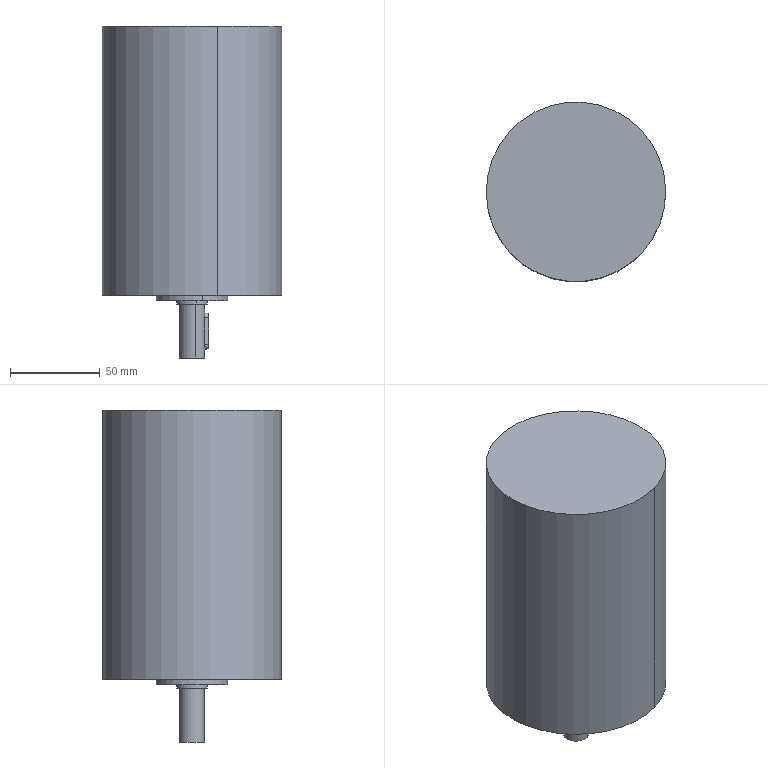Component | SolidWorks | DSEM-GDCServoGearMotor-1 | 1 solid | 35 faces | box 100 x 100 x 185 mm | volume 1186432 mm3 | cylinder 19 | cone 8 | plane 8 | commonest cylinder face diameters 4.2 x8 5 x3 40 x2 17 x2 100 x2 14 x2
build123d program:
from build123d import *

# Parameters (mm, degrees)
CIRPATTERN2_COUNT   = 4
BOSS_EXTRUDE1_DEPTH = 9


with BuildPart() as part:
    # Sketch1 → Revolve2 (revolve)
    with BuildSketch(Plane(origin=(0, 0, 0), x_dir=(0, 0, -1), z_dir=(1, 0, 0)), mode=Mode.PRIVATE) as revolve2_sk:
        Polygon((0, 20), (0, 50), (150, 50), (150, 0), (-35, 0), (-35, 7), (-5, 7), (-5, 8.5), (-3, 8.5), (-3, 20), align=None)
    revolve(revolve2_sk.sketch.rotate(Axis((0, 0, 38.169), (0, 0, -1)), 90), axis=Axis((0, 0, 38.169), (0, 0, -1)))

    # Sketch7 → M5 Tapped Hole2 (revolve, cut)
    with BuildSketch(Plane(origin=(-18.385, 18.385, 0), x_dir=(0, -1, 0), z_dir=(1, 0, 0))):
        Polygon((0, 0), (0, 13.662), (2.1, 12.4), (2.1, 0), align=None)
    m5_tapped_hole2 = revolve(axis=Axis((-18.385, 18.385, 6.35), (0, 0, -1)), mode=Mode.SUBTRACT)

    # CirPattern2: M5 Tapped Hole2 ×4 about axis
    cirpattern2_axis = Axis((0, 0, 0), (0, 0, 1))
    for i in range(1, CIRPATTERN2_COUNT):
        add(m5_tapped_hole2.rotate(cirpattern2_axis, i * 360 / CIRPATTERN2_COUNT), mode=Mode.SUBTRACT)

    # Sketch9 → Boss-Extrude1 (add)
    with BuildSketch(Plane(origin=(0, 0, 0), x_dir=(1, 0, 0), z_dir=(0, 1, 0))):
        with BuildLine():
            Line((2.5, -12.5), (2.5, -27.5))
            ThreePointArc((2.5, -27.5), (0, -30), (-2.5, -27.5))
            Line((-2.5, -27.5), (-2.5, -12.5))
            ThreePointArc((-2.5, -12.5), (0, -10), (2.5, -12.5))
        make_face()
    extrude(amount=BOSS_EXTRUDE1_DEPTH)


solid = part.part

# Placed as in the assembly
solid = solid.moved(Location((25.629, -64.9, 271), (-180, 0, -106.616)))
STEP:
#1=COLOUR_RGB('',0.7922,0.8196,0.9333);
#2=FILL_AREA_STYLE_COLOUR('',#1);
#3=FILL_AREA_STYLE('',(#2));
#4=SURFACE_STYLE_FILL_AREA(#3);
#5=SURFACE_SIDE_STYLE('',(#4));
#6=SURFACE_STYLE_USAGE(.BOTH.,#5);
#7=PRESENTATION_STYLE_ASSIGNMENT((#6));
#8=CARTESIAN_POINT('',(1.349,-2.454,10.276));
#9=VERTEX_POINT('',#8);
#10=CARTESIAN_POINT('',(1.377,-2.548,10.177));
#11=VERTEX_POINT('',#10);
#12=CARTESIAN_POINT('',(1.349,-2.454,10.177));
#13=DIRECTION('',(0.9582,0.286,-0.));
#14=DIRECTION('',(0.,0.,-1.));
#15=AXIS2_PLACEMENT_3D('',#12,#13,#14);
#16=CIRCLE('',#15,0.09843);
#17=EDGE_CURVE('',#9,#11,#16,.T.);
#18=ORIENTED_EDGE('',*,*,#17,.F.);
#19=CARTESIAN_POINT('',(1.273,-2.476,10.276));
#20=VERTEX_POINT('',#19);
#21=CARTESIAN_POINT('',(1.349,-2.454,10.276));
#22=DIRECTION('',(-0.9582,-0.286,0.));
#23=VECTOR('',#22,39.37);
#24=LINE('',#21,#23);
#25=EDGE_CURVE('',#9,#20,#24,.T.);
#26=ORIENTED_EDGE('',*,*,#25,.T.);
#27=CARTESIAN_POINT('',(1.284,-2.576,10.177));
#28=VERTEX_POINT('',#27);
#29=CARTESIAN_POINT('',(1.273,-2.476,10.276));
#30=CARTESIAN_POINT('',(1.275,-2.483,10.276));
#31=CARTESIAN_POINT('',(1.277,-2.489,10.275));
#32=CARTESIAN_POINT('',(1.279,-2.501,10.272));
#33=CARTESIAN_POINT('',(1.281,-2.507,10.27));
#34=CARTESIAN_POINT('',(1.282,-2.519,10.266));
#35=CARTESIAN_POINT('',(1.283,-2.525,10.262));
#36=CARTESIAN_POINT('',(1.284,-2.536,10.255));
#37=CARTESIAN_POINT('',(1.284,-2.541,10.251));
#38=CARTESIAN_POINT('',(1.285,-2.555,10.238));
#39=CARTESIAN_POINT('',(1.285,-2.563,10.227));
#40=CARTESIAN_POINT('',(1.284,-2.57,10.209));
#41=CARTESIAN_POINT('',(1.284,-2.572,10.203));
#42=CARTESIAN_POINT('',(1.284,-2.575,10.19));
#43=CARTESIAN_POINT('',(1.284,-2.576,10.184));
#44=CARTESIAN_POINT('',(1.284,-2.576,10.177));
#45=B_SPLINE_CURVE_WITH_KNOTS('',3,(#29,#30,#31,#32,#33,#34,#35,#36,#37,#38,#39,#40,#41,#42,#43,#44),.UNSPECIFIED.,.F.,.F.,(4,2,2,2,2,2,2,4),(0.,0.0004928,0.0009856,0.001478,0.001971,0.002957,0.003449,0.003942),.UNSPECIFIED.);
#46=EDGE_CURVE('',#20,#28,#45,.T.);
#47=ORIENTED_EDGE('',*,*,#46,.T.);
#48=CARTESIAN_POINT('',(1.377,-2.548,10.177));
#49=DIRECTION('',(-0.9582,-0.286,0.));
#50=VECTOR('',#49,39.37);
#51=LINE('',#48,#50);
#52=EDGE_CURVE('',#11,#28,#51,.T.);
#53=ORIENTED_EDGE('',*,*,#52,.F.);
#54=EDGE_LOOP('',(#18,#26,#47,#53));
#55=FACE_OUTER_BOUND('',#54,.T.);
#56=CARTESIAN_POINT('',(1.349,-2.454,10.177));
#57=DIRECTION('',(-0.9582,-0.286,0.));
#58=DIRECTION('',(0.,0.,1.));
#59=AXIS2_PLACEMENT_3D('',#56,#57,#58);
#60=CYLINDRICAL_SURFACE('',#59,0.09843);
#61=ADVANCED_FACE('',(#55),#60,.T.);
#62=CARTESIAN_POINT('',(0.5461,-3.535,11.157));
#63=VERTEX_POINT('',#62);
#64=CARTESIAN_POINT('',(0.4988,-3.376,11.157));
#65=VERTEX_POINT('',#64);
#66=CARTESIAN_POINT('',(0.5224,-3.456,11.157));
#67=DIRECTION('',(-0.,0.,-1.));
#68=DIRECTION('',(-0.286,0.9582,0.));
#69=AXIS2_PLACEMENT_3D('',#66,#67,#68);
#70=CIRCLE('',#69,0.08268);
#71=EDGE_CURVE('',#63,#65,#70,.T.);
#72=ORIENTED_EDGE('',*,*,#71,.F.);
#73=CARTESIAN_POINT('',(0.5461,-3.535,10.669));
#74=VERTEX_POINT('',#73);
#75=CARTESIAN_POINT('',(0.5461,-3.535,10.669));
#76=DIRECTION('',(-0.,0.,-1.));
#77=VECTOR('',#76,39.37);
#78=LINE('',#75,#77);
#79=EDGE_CURVE('',#63,#74,#78,.T.);
#80=ORIENTED_EDGE('',*,*,#79,.T.);
#81=CARTESIAN_POINT('',(0.4988,-3.376,10.669));
#82=VERTEX_POINT('',#81);
#83=CARTESIAN_POINT('',(0.5224,-3.456,10.669));
#84=DIRECTION('',(-0.,0.,-1.));
#85=DIRECTION('',(-0.286,0.9582,0.));
#86=AXIS2_PLACEMENT_3D('',#83,#84,#85);
#87=CIRCLE('',#86,0.08268);
#88=EDGE_CURVE('',#74,#82,#87,.T.);
#89=ORIENTED_EDGE('',*,*,#88,.T.);
#90=CARTESIAN_POINT('',(0.4988,-3.376,10.669));
#91=DIRECTION('',(-0.,0.,-1.));
#92=VECTOR('',#91,39.37);
#93=LINE('',#90,#92);
#94=EDGE_CURVE('',#65,#82,#93,.T.);
#95=ORIENTED_EDGE('',*,*,#94,.F.);
#96=EDGE_LOOP('',(#72,#80,#89,#95));
#97=FACE_OUTER_BOUND('',#96,.T.);
#98=CARTESIAN_POINT('',(0.5224,-3.456,10.669));
#99=DIRECTION('',(-0.,0.,-1.));
#100=DIRECTION('',(-0.286,0.9582,0.));
#101=AXIS2_PLACEMENT_3D('',#98,#99,#100);
#102=CYLINDRICAL_SURFACE('',#101,0.08268);
#103=ADVANCED_FACE('',(#97),#102,.F.);
#104=CARTESIAN_POINT('',(0.5224,-3.456,11.207));
#105=VERTEX_POINT('',#104);
#106=CARTESIAN_POINT('',(0.4988,-3.376,11.157));
#107=DIRECTION('',(-0.2451,0.8214,-0.515));
#108=VECTOR('',#107,39.37);
#109=LINE('',#106,#108);
#110=EDGE_CURVE('',#105,#65,#109,.T.);
#111=ORIENTED_EDGE('',*,*,#110,.F.);
#112=CARTESIAN_POINT('',(0.5461,-3.535,11.157));
#113=DIRECTION('',(0.2451,-0.8214,-0.515));
#114=VECTOR('',#113,39.37);
#115=LINE('',#112,#114);
#116=EDGE_CURVE('',#105,#63,#115,.T.);
#117=ORIENTED_EDGE('',*,*,#116,.T.);
#118=ORIENTED_EDGE('',*,*,#71,.T.);
#119=EDGE_LOOP('',(#111,#117,#118));
#120=FACE_OUTER_BOUND('',#119,.T.);
#121=CARTESIAN_POINT('',(0.5224,-3.456,11.157));
#122=DIRECTION('',(-0.,0.,-1.));
#123=DIRECTION('',(-0.286,0.9582,0.));
#124=AXIS2_PLACEMENT_3D('',#121,#122,#123);
#125=CONICAL_SURFACE('',#124,0.08268,1.03);
#126=ADVANCED_FACE('',(#120),#125,.F.);
#127=CARTESIAN_POINT('',(0.1321,-2.148,11.157));
#128=VERTEX_POINT('',#127);
#129=CARTESIAN_POINT('',(0.08483,-1.989,11.157));
#130=VERTEX_POINT('',#129);
#131=CARTESIAN_POINT('',(0.1085,-2.069,11.157));
#132=DIRECTION('',(-0.,0.,-1.));
#133=DIRECTION('',(-0.286,0.9582,0.));
#134=AXIS2_PLACEMENT_3D('',#131,#132,#133);
#135=CIRCLE('',#134,0.08268);
#136=EDGE_CURVE('',#128,#130,#135,.T.);
#137=ORIENTED_EDGE('',*,*,#136,.F.);
#138=CARTESIAN_POINT('',(0.1321,-2.148,10.669));
#139=VERTEX_POINT('',#138);
#140=CARTESIAN_POINT('',(0.1321,-2.148,10.669));
#141=DIRECTION('',(-0.,0.,-1.));
#142=VECTOR('',#141,39.37);
#143=LINE('',#140,#142);
#144=EDGE_CURVE('',#128,#139,#143,.T.);
#145=ORIENTED_EDGE('',*,*,#144,.T.);
#146=CARTESIAN_POINT('',(0.08483,-1.989,10.669));
#147=VERTEX_POINT('',#146);
#148=CARTESIAN_POINT('',(0.1085,-2.069,10.669));
#149=DIRECTION('',(-0.,0.,-1.));
#150=DIRECTION('',(-0.286,0.9582,0.));
#151=AXIS2_PLACEMENT_3D('',#148,#149,#150);
#152=CIRCLE('',#151,0.08268);
#153=EDGE_CURVE('',#139,#147,#152,.T.);
#154=ORIENTED_EDGE('',*,*,#153,.T.);
#155=CARTESIAN_POINT('',(0.08483,-1.989,10.669));
#156=DIRECTION('',(-0.,0.,-1.));
#157=VECTOR('',#156,39.37);
#158=LINE('',#155,#157);
#159=EDGE_CURVE('',#130,#147,#158,.T.);
#160=ORIENTED_EDGE('',*,*,#159,.F.);
#161=EDGE_LOOP('',(#137,#145,#154,#160));
#162=FACE_OUTER_BOUND('',#161,.T.);
#163=CARTESIAN_POINT('',(0.1085,-2.069,10.669));
#164=DIRECTION('',(-0.,0.,-1.));
#165=DIRECTION('',(-0.286,0.9582,0.));
#166=AXIS2_PLACEMENT_3D('',#163,#164,#165);
#167=CYLINDRICAL_SURFACE('',#166,0.08268);
#168=ADVANCED_FACE('',(#162),#167,.F.);
#169=CARTESIAN_POINT('',(0.1085,-2.069,11.207));
#170=VERTEX_POINT('',#169);
#171=CARTESIAN_POINT('',(0.08483,-1.989,11.157));
#172=DIRECTION('',(-0.2451,0.8214,-0.515));
#173=VECTOR('',#172,39.37);
#174=LINE('',#171,#173);
#175=EDGE_CURVE('',#170,#130,#174,.T.);
#176=ORIENTED_EDGE('',*,*,#175,.F.);
#177=CARTESIAN_POINT('',(0.1321,-2.148,11.157));
#178=DIRECTION('',(0.2451,-0.8214,-0.515));
#179=VECTOR('',#178,39.37);
#180=LINE('',#177,#179);
#181=EDGE_CURVE('',#170,#128,#180,.T.);
#182=ORIENTED_EDGE('',*,*,#181,.T.);
#183=ORIENTED_EDGE('',*,*,#136,.T.);
#184=EDGE_LOOP('',(#176,#182,#183));
#185=FACE_OUTER_BOUND('',#184,.T.);
#186=CARTESIAN_POINT('',(0.1085,-2.069,11.157));
#187=DIRECTION('',(-0.,0.,-1.));
#188=DIRECTION('',(-0.286,0.9582,0.));
#189=AXIS2_PLACEMENT_3D('',#186,#187,#188);
#190=CONICAL_SURFACE('',#189,0.08268,1.03);
#191=ADVANCED_FACE('',(#185),#190,.F.);
#192=CARTESIAN_POINT('',(1.519,-1.734,11.157));
#193=VERTEX_POINT('',#192);
#194=CARTESIAN_POINT('',(1.472,-1.575,11.157));
#195=VERTEX_POINT('',#194);
#196=CARTESIAN_POINT('',(1.496,-1.655,11.157));
#197=DIRECTION('',(-0.,0.,-1.));
#198=DIRECTION('',(-0.286,0.9582,0.));
#199=AXIS2_PLACEMENT_3D('',#196,#197,#198);
#200=CIRCLE('',#199,0.08268);
#201=EDGE_CURVE('',#193,#195,#200,.T.);
#202=ORIENTED_EDGE('',*,*,#201,.F.);
#203=CARTESIAN_POINT('',(1.519,-1.734,10.669));
#204=VERTEX_POINT('',#203);
#205=CARTESIAN_POINT('',(1.519,-1.734,10.669));
#206=DIRECTION('',(-0.,0.,-1.));
#207=VECTOR('',#206,39.37);
#208=LINE('',#205,#207);
#209=EDGE_CURVE('',#193,#204,#208,.T.);
#210=ORIENTED_EDGE('',*,*,#209,.T.);
#211=CARTESIAN_POINT('',(1.472,-1.575,10.669));
#212=VERTEX_POINT('',#211);
#213=CARTESIAN_POINT('',(1.496,-1.655,10.669));
#214=DIRECTION('',(-0.,0.,-1.));
#215=DIRECTION('',(-0.286,0.9582,0.));
#216=AXIS2_PLACEMENT_3D('',#213,#214,#215);
#217=CIRCLE('',#216,0.08268);
#218=EDGE_CURVE('',#204,#212,#217,.T.);
#219=ORIENTED_EDGE('',*,*,#218,.T.);
#220=CARTESIAN_POINT('',(1.472,-1.575,10.669));
#221=DIRECTION('',(-0.,0.,-1.));
#222=VECTOR('',#221,39.37);
#223=LINE('',#220,#222);
#224=EDGE_CURVE('',#195,#212,#223,.T.);
#225=ORIENTED_EDGE('',*,*,#224,.F.);
#226=EDGE_LOOP('',(#202,#210,#219,#225));
#227=FACE_OUTER_BOUND('',#226,.T.);
#228=CARTESIAN_POINT('',(1.496,-1.655,10.669));
#229=DIRECTION('',(-0.,0.,-1.));
#230=DIRECTION('',(-0.286,0.9582,0.));
#231=AXIS2_PLACEMENT_3D('',#228,#229,#230);
#232=CYLINDRICAL_SURFACE('',#231,0.08268);
#233=ADVANCED_FACE('',(#227),#232,.F.);
#234=CARTESIAN_POINT('',(1.496,-1.655,11.207));
#235=VERTEX_POINT('',#234);
#236=CARTESIAN_POINT('',(1.472,-1.575,11.157));
#237=DIRECTION('',(-0.2451,0.8214,-0.515));
#238=VECTOR('',#237,39.37);
#239=LINE('',#236,#238);
#240=EDGE_CURVE('',#235,#195,#239,.T.);
#241=ORIENTED_EDGE('',*,*,#240,.F.);
#242=CARTESIAN_POINT('',(1.519,-1.734,11.157));
#243=DIRECTION('',(0.2451,-0.8214,-0.515));
#244=VECTOR('',#243,39.37);
#245=LINE('',#242,#244);
#246=EDGE_CURVE('',#235,#193,#245,.T.);
#247=ORIENTED_EDGE('',*,*,#246,.T.);
#248=ORIENTED_EDGE('',*,*,#201,.T.);
#249=EDGE_LOOP('',(#241,#247,#248));
#250=FACE_OUTER_BOUND('',#249,.T.);
#251=CARTESIAN_POINT('',(1.496,-1.655,11.157));
#252=DIRECTION('',(-0.,0.,-1.));
#253=DIRECTION('',(-0.286,0.9582,0.));
#254=AXIS2_PLACEMENT_3D('',#251,#252,#253);
#255=CONICAL_SURFACE('',#254,0.08268,1.03);
#256=ADVANCED_FACE('',(#250),#255,.F.);
#257=CARTESIAN_POINT('',(1.933,-3.121,11.157));
#258=VERTEX_POINT('',#257);
#259=CARTESIAN_POINT('',(1.886,-2.963,11.157));
#260=VERTEX_POINT('',#259);
#261=CARTESIAN_POINT('',(1.91,-3.042,11.157));
#262=DIRECTION('',(-0.,0.,-1.));
#263=DIRECTION('',(-0.286,0.9582,0.));
#264=AXIS2_PLACEMENT_3D('',#261,#262,#263);
#265=CIRCLE('',#264,0.08268);
#266=EDGE_CURVE('',#258,#260,#265,.T.);
#267=ORIENTED_EDGE('',*,*,#266,.F.);
#268=CARTESIAN_POINT('',(1.933,-3.121,10.669));
#269=VERTEX_POINT('',#268);
#270=CARTESIAN_POINT('',(1.933,-3.121,10.669));
#271=DIRECTION('',(-0.,0.,-1.));
#272=VECTOR('',#271,39.37);
#273=LINE('',#270,#272);
#274=EDGE_CURVE('',#258,#269,#273,.T.);
#275=ORIENTED_EDGE('',*,*,#274,.T.);
#276=CARTESIAN_POINT('',(1.886,-2.963,10.669));
#277=VERTEX_POINT('',#276);
#278=CARTESIAN_POINT('',(1.91,-3.042,10.669));
#279=DIRECTION('',(-0.,0.,-1.));
#280=DIRECTION('',(-0.286,0.9582,0.));
#281=AXIS2_PLACEMENT_3D('',#278,#279,#280);
#282=CIRCLE('',#281,0.08268);
#283=EDGE_CURVE('',#269,#277,#282,.T.);
#284=ORIENTED_EDGE('',*,*,#283,.T.);
#285=CARTESIAN_POINT('',(1.886,-2.963,10.669));
#286=DIRECTION('',(-0.,0.,-1.));
#287=VECTOR('',#286,39.37);
#288=LINE('',#285,#287);
#289=EDGE_CURVE('',#260,#277,#288,.T.);
#290=ORIENTED_EDGE('',*,*,#289,.F.);
#291=EDGE_LOOP('',(#267,#275,#284,#290));
#292=FACE_OUTER_BOUND('',#291,.T.);
#293=CARTESIAN_POINT('',(1.91,-3.042,10.669));
#294=DIRECTION('',(-0.,0.,-1.));
#295=DIRECTION('',(-0.286,0.9582,0.));
#296=AXIS2_PLACEMENT_3D('',#293,#294,#295);
#297=CYLINDRICAL_SURFACE('',#296,0.08268);
#298=ADVANCED_FACE('',(#292),#297,.F.);
#299=CARTESIAN_POINT('',(1.91,-3.042,11.207));
#300=VERTEX_POINT('',#299);
#301=CARTESIAN_POINT('',(1.886,-2.963,11.157));
#302=DIRECTION('',(-0.2451,0.8214,-0.515));
#303=VECTOR('',#302,39.37);
#304=LINE('',#301,#303);
#305=EDGE_CURVE('',#300,#260,#304,.T.);
#306=ORIENTED_EDGE('',*,*,#305,.F.);
#307=CARTESIAN_POINT('',(1.933,-3.121,11.157));
#308=DIRECTION('',(0.2451,-0.8214,-0.515));
#309=VECTOR('',#308,39.37);
#310=LINE('',#307,#309);
#311=EDGE_CURVE('',#300,#258,#310,.T.);
#312=ORIENTED_EDGE('',*,*,#311,.T.);
#313=ORIENTED_EDGE('',*,*,#266,.T.);
#314=EDGE_LOOP('',(#306,#312,#313));
#315=FACE_OUTER_BOUND('',#314,.T.);
#316=CARTESIAN_POINT('',(1.91,-3.042,11.157));
#317=DIRECTION('',(-0.,0.,-1.));
#318=DIRECTION('',(-0.286,0.9582,0.));
#319=AXIS2_PLACEMENT_3D('',#316,#317,#318);
#320=CONICAL_SURFACE('',#319,0.08268,1.03);
#321=ADVANCED_FACE('',(#315),#320,.F.);
#322=CARTESIAN_POINT('',(0.7839,-1.801,10.669));
#323=VERTEX_POINT('',#322);
#324=CARTESIAN_POINT('',(1.234,-3.31,10.669));
#325=VERTEX_POINT('',#324);
#326=CARTESIAN_POINT('',(1.009,-2.555,10.669));
#327=DIRECTION('',(-0.,0.,-1.));
#328=DIRECTION('',(-0.286,0.9582,0.));
#329=AXIS2_PLACEMENT_3D('',#326,#327,#328);
#330=CIRCLE('',#329,0.7874);
#331=EDGE_CURVE('',#323,#325,#330,.T.);
#332=ORIENTED_EDGE('',*,*,#331,.T.);
#333=CARTESIAN_POINT('',(1.234,-3.31,10.551));
#334=VERTEX_POINT('',#333);
#335=CARTESIAN_POINT('',(1.234,-3.31,9.167));
#336=DIRECTION('',(-0.,0.,-1.));
#337=VECTOR('',#336,39.37);
#338=LINE('',#335,#337);
#339=EDGE_CURVE('',#325,#334,#338,.T.);
#340=ORIENTED_EDGE('',*,*,#339,.T.);
#341=CARTESIAN_POINT('',(0.7839,-1.801,10.551));
#342=VERTEX_POINT('',#341);
#343=CARTESIAN_POINT('',(1.009,-2.555,10.551));
#344=DIRECTION('',(-0.,0.,-1.));
#345=DIRECTION('',(-0.286,0.9582,0.));
#346=AXIS2_PLACEMENT_3D('',#343,#344,#345);
#347=CIRCLE('',#346,0.7874);
#348=EDGE_CURVE('',#342,#334,#347,.T.);
#349=ORIENTED_EDGE('',*,*,#348,.F.);
#350=CARTESIAN_POINT('',(0.7839,-1.801,9.167));
#351=DIRECTION('',(-0.,0.,-1.));
#352=VECTOR('',#351,39.37);
#353=LINE('',#350,#352);
#354=EDGE_CURVE('',#323,#342,#353,.T.);
#355=ORIENTED_EDGE('',*,*,#354,.F.);
#356=EDGE_LOOP('',(#332,#340,#349,#355));
#357=FACE_OUTER_BOUND('',#356,.T.);
#358=CARTESIAN_POINT('',(1.009,-2.555,9.167));
#359=DIRECTION('',(-0.,0.,-1.));
#360=DIRECTION('',(-0.286,0.9582,0.));
#361=AXIS2_PLACEMENT_3D('',#358,#359,#360);
#362=CYLINDRICAL_SURFACE('',#361,0.7874);
#363=ADVANCED_FACE('',(#357),#362,.T.);
#364=CARTESIAN_POINT('',(0.9133,-2.234,10.551));
#365=VERTEX_POINT('',#364);
#366=CARTESIAN_POINT('',(1.105,-2.876,10.551));
#367=VERTEX_POINT('',#366);
#368=CARTESIAN_POINT('',(1.009,-2.555,10.551));
#369=DIRECTION('',(-0.,0.,-1.));
#370=DIRECTION('',(-0.286,0.9582,0.));
#371=AXIS2_PLACEMENT_3D('',#368,#369,#370);
#372=CIRCLE('',#371,0.3346);
#373=EDGE_CURVE('',#365,#367,#372,.T.);
#374=ORIENTED_EDGE('',*,*,#373,.T.);
#375=CARTESIAN_POINT('',(1.105,-2.876,10.472));
#376=VERTEX_POINT('',#375);
#377=CARTESIAN_POINT('',(1.105,-2.876,9.167));
#378=DIRECTION('',(-0.,0.,-1.));
#379=VECTOR('',#378,39.37);
#380=LINE('',#377,#379);
#381=EDGE_CURVE('',#367,#376,#380,.T.);
#382=ORIENTED_EDGE('',*,*,#381,.T.);
#383=CARTESIAN_POINT('',(0.9133,-2.234,10.472));
#384=VERTEX_POINT('',#383);
#385=CARTESIAN_POINT('',(1.009,-2.555,10.472));
#386=DIRECTION('',(-0.,0.,-1.));
#387=DIRECTION('',(-0.286,0.9582,0.));
#388=AXIS2_PLACEMENT_3D('',#385,#386,#387);
#389=CIRCLE('',#388,0.3346);
#390=EDGE_CURVE('',#384,#376,#389,.T.);
#391=ORIENTED_EDGE('',*,*,#390,.F.);
#392=CARTESIAN_POINT('',(0.9133,-2.234,9.167));
#393=DIRECTION('',(-0.,0.,-1.));
#394=VECTOR('',#393,39.37);
#395=LINE('',#392,#394);
#396=EDGE_CURVE('',#365,#384,#395,.T.);
#397=ORIENTED_EDGE('',*,*,#396,.F.);
#398=EDGE_LOOP('',(#374,#382,#391,#397));
#399=FACE_OUTER_BOUND('',#398,.T.);
#400=CARTESIAN_POINT('',(1.009,-2.555,9.167));
#401=DIRECTION('',(-0.,0.,-1.));
#402=DIRECTION('',(-0.286,0.9582,0.));
#403=AXIS2_PLACEMENT_3D('',#400,#401,#402);
#404=CYLINDRICAL_SURFACE('',#403,0.3346);
#405=ADVANCED_FACE('',(#399),#404,.T.);
#406=CARTESIAN_POINT('',(0.4461,-0.6688,16.575));
#407=VERTEX_POINT('',#406);
#408=CARTESIAN_POINT('',(1.572,-4.441,16.575));
#409=VERTEX_POINT('',#408);
#410=CARTESIAN_POINT('',(1.009,-2.555,16.575));
#411=DIRECTION('',(-0.,0.,-1.));
#412=DIRECTION('',(-0.286,0.9582,0.));
#413=AXIS2_PLACEMENT_3D('',#410,#411,#412);
#414=CIRCLE('',#413,1.969);
#415=EDGE_CURVE('',#407,#409,#414,.T.);
#416=ORIENTED_EDGE('',*,*,#415,.T.);
#417=CARTESIAN_POINT('',(1.572,-4.441,10.669));
#418=VERTEX_POINT('',#417);
#419=CARTESIAN_POINT('',(1.572,-4.441,9.167));
#420=DIRECTION('',(-0.,0.,-1.));
#421=VECTOR('',#420,39.37);
#422=LINE('',#419,#421);
#423=EDGE_CURVE('',#409,#418,#422,.T.);
#424=ORIENTED_EDGE('',*,*,#423,.T.);
#425=CARTESIAN_POINT('',(0.4461,-0.6688,10.669));
#426=VERTEX_POINT('',#425);
#427=CARTESIAN_POINT('',(1.009,-2.555,10.669));
#428=DIRECTION('',(-0.,0.,-1.));
#429=DIRECTION('',(-0.286,0.9582,0.));
#430=AXIS2_PLACEMENT_3D('',#427,#428,#429);
#431=CIRCLE('',#430,1.969);
#432=EDGE_CURVE('',#426,#418,#431,.T.);
#433=ORIENTED_EDGE('',*,*,#432,.F.);
#434=CARTESIAN_POINT('',(0.4461,-0.6688,9.167));
#435=DIRECTION('',(-0.,0.,-1.));
#436=VECTOR('',#435,39.37);
#437=LINE('',#434,#436);
#438=EDGE_CURVE('',#407,#426,#437,.T.);
#439=ORIENTED_EDGE('',*,*,#438,.F.);
#440=EDGE_LOOP('',(#416,#424,#433,#439));
#441=FACE_OUTER_BOUND('',#440,.T.);
#442=CARTESIAN_POINT('',(1.009,-2.555,9.167));
#443=DIRECTION('',(-0.,0.,-1.));
#444=DIRECTION('',(-0.286,0.9582,0.));
#445=AXIS2_PLACEMENT_3D('',#442,#443,#444);
#446=CYLINDRICAL_SURFACE('',#445,1.969);
#447=ADVANCED_FACE('',(#441),#446,.T.);
#448=CARTESIAN_POINT('',(1.228,-2.387,10.177));
#449=VERTEX_POINT('',#448);
#450=CARTESIAN_POINT('',(1.228,-2.387,10.177));
#451=CARTESIAN_POINT('',(1.228,-2.387,10.184));
#452=CARTESIAN_POINT('',(1.228,-2.388,10.19));
#453=CARTESIAN_POINT('',(1.23,-2.39,10.203));
#454=CARTESIAN_POINT('',(1.231,-2.392,10.209));
#455=CARTESIAN_POINT('',(1.234,-2.396,10.221));
#456=CARTESIAN_POINT('',(1.236,-2.398,10.227));
#457=CARTESIAN_POINT('',(1.24,-2.405,10.237));
#458=CARTESIAN_POINT('',(1.242,-2.408,10.242));
#459=CARTESIAN_POINT('',(1.247,-2.416,10.251));
#460=CARTESIAN_POINT('',(1.25,-2.421,10.255));
#461=CARTESIAN_POINT('',(1.255,-2.43,10.263));
#462=CARTESIAN_POINT('',(1.257,-2.435,10.266));
#463=CARTESIAN_POINT('',(1.262,-2.446,10.271));
#464=CARTESIAN_POINT('',(1.265,-2.452,10.272));
#465=CARTESIAN_POINT('',(1.269,-2.464,10.275));
#466=CARTESIAN_POINT('',(1.271,-2.47,10.276));
#467=CARTESIAN_POINT('',(1.273,-2.476,10.276));
#468=B_SPLINE_CURVE_WITH_KNOTS('',3,(#450,#451,#452,#453,#454,#455,#456,#457,#458,#459,#460,#461,#462,#463,#464,#465,#466,#467),.UNSPECIFIED.,.F.,.F.,(4,2,2,2,2,2,2,2,4),(0.01182,0.01231,0.01281,0.0133,0.01379,0.01428,0.01478,0.01527,0.01576),.UNSPECIFIED.);
#469=EDGE_CURVE('',#449,#20,#468,.T.);
#470=ORIENTED_EDGE('',*,*,#469,.F.);
#471=CARTESIAN_POINT('',(1.228,-2.387,9.587));
#472=VERTEX_POINT('',#471);
#473=CARTESIAN_POINT('',(1.228,-2.387,9.167));
#474=DIRECTION('',(0.,-0.,1.));
#475=VECTOR('',#474,39.37);
#476=LINE('',#473,#475);
#477=EDGE_CURVE('',#472,#449,#476,.T.);
#478=ORIENTED_EDGE('',*,*,#477,.F.);
#479=CARTESIAN_POINT('',(1.284,-2.576,9.587));
#480=VERTEX_POINT('',#479);
#481=CARTESIAN_POINT('',(1.284,-2.576,9.587));
#482=CARTESIAN_POINT('',(1.284,-2.576,9.58));
#483=CARTESIAN_POINT('',(1.284,-2.575,9.574));
#484=CARTESIAN_POINT('',(1.284,-2.572,9.561));
#485=CARTESIAN_POINT('',(1.284,-2.57,9.555));
#486=CARTESIAN_POINT('',(1.284,-2.565,9.543));
#487=CARTESIAN_POINT('',(1.285,-2.562,9.537));
#488=CARTESIAN_POINT('',(1.285,-2.554,9.526));
#489=CARTESIAN_POINT('',(1.285,-2.55,9.521));
#490=CARTESIAN_POINT('',(1.284,-2.541,9.512));
#491=CARTESIAN_POINT('',(1.284,-2.536,9.508));
#492=CARTESIAN_POINT('',(1.283,-2.525,9.501));
#493=CARTESIAN_POINT('',(1.282,-2.519,9.498));
#494=CARTESIAN_POINT('',(1.281,-2.507,9.493));
#495=CARTESIAN_POINT('',(1.279,-2.501,9.491));
#496=CARTESIAN_POINT('',(1.277,-2.489,9.489));
#497=CARTESIAN_POINT('',(1.275,-2.483,9.488));
#498=CARTESIAN_POINT('',(1.271,-2.47,9.488));
#499=CARTESIAN_POINT('',(1.269,-2.464,9.489));
#500=CARTESIAN_POINT('',(1.265,-2.452,9.491));
#501=CARTESIAN_POINT('',(1.262,-2.446,9.493));
#502=CARTESIAN_POINT('',(1.257,-2.435,9.498));
#503=CARTESIAN_POINT('',(1.255,-2.43,9.501));
#504=CARTESIAN_POINT('',(1.25,-2.421,9.508));
#505=CARTESIAN_POINT('',(1.247,-2.416,9.512));
#506=CARTESIAN_POINT('',(1.242,-2.408,9.522));
#507=CARTESIAN_POINT('',(1.24,-2.405,9.527));
#508=CARTESIAN_POINT('',(1.236,-2.398,9.537));
#509=CARTESIAN_POINT('',(1.234,-2.396,9.543));
#510=CARTESIAN_POINT('',(1.231,-2.392,9.555));
#511=CARTESIAN_POINT('',(1.23,-2.39,9.561));
#512=CARTESIAN_POINT('',(1.228,-2.388,9.574));
#513=CARTESIAN_POINT('',(1.228,-2.387,9.58));
#514=CARTESIAN_POINT('',(1.228,-2.387,9.587));
#515=B_SPLINE_CURVE_WITH_KNOTS('',3,(#481,#482,#483,#484,#485,#486,#487,#488,#489,#490,#491,#492,#493,#494,#495,#496,#497,#498,#499,#500,#501,#502,#503,#504,#505,#506,#507,#508,#509,#510,#511,#512,#513,#514),.UNSPECIFIED.,.F.,.F.,(4,2,2,2,2,2,2,2,2,2,2,2,2,2,2,2,4),(0.003942,0.004435,0.004927,0.005419,0.005912,0.006404,0.006897,0.007389,0.007882,0.008374,0.008866,0.009359,0.009851,0.01034,0.01084,0.01133,0.01182),.UNSPECIFIED.);
#516=EDGE_CURVE('',#480,#472,#515,.T.);
#517=ORIENTED_EDGE('',*,*,#516,.F.);
#518=CARTESIAN_POINT('',(1.284,-2.576,9.167));
#519=DIRECTION('',(-0.,0.,-1.));
#520=VECTOR('',#519,39.37);
#521=LINE('',#518,#520);
#522=EDGE_CURVE('',#28,#480,#521,.T.);
#523=ORIENTED_EDGE('',*,*,#522,.F.);
#524=ORIENTED_EDGE('',*,*,#46,.F.);
#525=EDGE_LOOP('',(#470,#478,#517,#523,#524));
#526=FACE_BOUND('',#525,.T.);
#527=CARTESIAN_POINT('',(0.9302,-2.291,10.472));
#528=VERTEX_POINT('',#527);
#529=CARTESIAN_POINT('',(1.088,-2.819,10.472));
#530=VERTEX_POINT('',#529);
#531=CARTESIAN_POINT('',(1.009,-2.555,10.472));
#532=DIRECTION('',(-0.,0.,-1.));
#533=DIRECTION('',(-0.286,0.9582,0.));
#534=AXIS2_PLACEMENT_3D('',#531,#532,#533);
#535=CIRCLE('',#534,0.2756);
#536=EDGE_CURVE('',#528,#530,#535,.T.);
#537=ORIENTED_EDGE('',*,*,#536,.T.);
#538=CARTESIAN_POINT('',(1.088,-2.819,9.291));
#539=VERTEX_POINT('',#538);
#540=CARTESIAN_POINT('',(1.088,-2.819,9.167));
#541=DIRECTION('',(-0.,0.,-1.));
#542=VECTOR('',#541,39.37);
#543=LINE('',#540,#542);
#544=EDGE_CURVE('',#530,#539,#543,.T.);
#545=ORIENTED_EDGE('',*,*,#544,.T.);
#546=CARTESIAN_POINT('',(0.9302,-2.291,9.291));
#547=VERTEX_POINT('',#546);
#548=CARTESIAN_POINT('',(1.009,-2.555,9.291));
#549=DIRECTION('',(-0.,0.,-1.));
#550=DIRECTION('',(-0.286,0.9582,0.));
#551=AXIS2_PLACEMENT_3D('',#548,#549,#550);
#552=CIRCLE('',#551,0.2756);
#553=EDGE_CURVE('',#547,#539,#552,.T.);
#554=ORIENTED_EDGE('',*,*,#553,.F.);
#555=CARTESIAN_POINT('',(0.9302,-2.291,9.167));
#556=DIRECTION('',(-0.,0.,-1.));
#557=VECTOR('',#556,39.37);
#558=LINE('',#555,#557);
#559=EDGE_CURVE('',#528,#547,#558,.T.);
#560=ORIENTED_EDGE('',*,*,#559,.F.);
#561=EDGE_LOOP('',(#537,#545,#554,#560));
#562=FACE_OUTER_BOUND('',#561,.T.);
#563=CARTESIAN_POINT('',(1.009,-2.555,9.167));
#564=DIRECTION('',(-0.,0.,-1.));
#565=DIRECTION('',(-0.286,0.9582,0.));
#566=AXIS2_PLACEMENT_3D('',#563,#564,#565);
#567=CYLINDRICAL_SURFACE('',#566,0.2756);
#568=ADVANCED_FACE('',(#526,#562),#567,.T.);
#569=ORIENTED_EDGE('',*,*,#544,.F.);
#570=CARTESIAN_POINT('',(1.009,-2.555,10.472));
#571=DIRECTION('',(-0.,0.,-1.));
#572=DIRECTION('',(-0.286,0.9582,0.));
#573=AXIS2_PLACEMENT_3D('',#570,#571,#572);
#574=CIRCLE('',#573,0.2756);
#575=EDGE_CURVE('',#530,#528,#574,.T.);
#576=ORIENTED_EDGE('',*,*,#575,.T.);
#577=ORIENTED_EDGE('',*,*,#559,.T.);
#578=CARTESIAN_POINT('',(1.009,-2.555,9.291));
#579=DIRECTION('',(-0.,0.,-1.));
#580=DIRECTION('',(-0.286,0.9582,0.));
#581=AXIS2_PLACEMENT_3D('',#578,#579,#580);
#582=CIRCLE('',#581,0.2756);
#583=EDGE_CURVE('',#539,#547,#582,.T.);
#584=ORIENTED_EDGE('',*,*,#583,.F.);
#585=EDGE_LOOP('',(#569,#576,#577,#584));
#586=FACE_OUTER_BOUND('',#585,.T.);
#587=CARTESIAN_POINT('',(1.009,-2.555,9.167));
#588=DIRECTION('',(-0.,0.,-1.));
#589=DIRECTION('',(-0.286,0.9582,0.));
#590=AXIS2_PLACEMENT_3D('',#587,#588,#589);
#591=CYLINDRICAL_SURFACE('',#590,0.2756);
#592=ADVANCED_FACE('',(#586),#591,.T.);
#593=ORIENTED_EDGE('',*,*,#423,.F.);
#594=CARTESIAN_POINT('',(1.009,-2.555,16.575));
#595=DIRECTION('',(-0.,0.,-1.));
#596=DIRECTION('',(-0.286,0.9582,0.));
#597=AXIS2_PLACEMENT_3D('',#594,#595,#596);
#598=CIRCLE('',#597,1.969);
#599=EDGE_CURVE('',#409,#407,#598,.T.);
#600=ORIENTED_EDGE('',*,*,#599,.T.);
#601=ORIENTED_EDGE('',*,*,#438,.T.);
#602=CARTESIAN_POINT('',(1.009,-2.555,10.669));
#603=DIRECTION('',(-0.,0.,-1.));
#604=DIRECTION('',(-0.286,0.9582,0.));
#605=AXIS2_PLACEMENT_3D('',#602,#603,#604);
#606=CIRCLE('',#605,1.969);
#607=EDGE_CURVE('',#418,#426,#606,.T.);
#608=ORIENTED_EDGE('',*,*,#607,.F.);
#609=EDGE_LOOP('',(#593,#600,#601,#608));
#610=FACE_OUTER_BOUND('',#609,.T.);
#611=CARTESIAN_POINT('',(1.009,-2.555,9.167));
#612=DIRECTION('',(-0.,0.,-1.));
#613=DIRECTION('',(-0.286,0.9582,0.));
#614=AXIS2_PLACEMENT_3D('',#611,#612,#613);
#615=CYLINDRICAL_SURFACE('',#614,1.969);
#616=ADVANCED_FACE('',(#610),#615,.T.);
#617=ORIENTED_EDGE('',*,*,#415,.F.);
#618=ORIENTED_EDGE('',*,*,#599,.F.);
#619=EDGE_LOOP('',(#617,#618));
#620=FACE_OUTER_BOUND('',#619,.T.);
#621=CARTESIAN_POINT('',(2.895,-1.992,16.575));
#622=DIRECTION('',(-0.,0.,-1.));
#623=DIRECTION('',(-0.286,0.9582,0.));
#624=AXIS2_PLACEMENT_3D('',#621,#622,#623);
#625=PLANE('',#624);
#626=ADVANCED_FACE('',(#620),#625,.F.);
#627=ORIENTED_EDGE('',*,*,#553,.T.);
#628=ORIENTED_EDGE('',*,*,#583,.T.);
#629=EDGE_LOOP('',(#627,#628));
#630=FACE_OUTER_BOUND('',#629,.T.);
#631=CARTESIAN_POINT('',(1.273,-2.476,9.291));
#632=DIRECTION('',(0.,-0.,1.));
#633=DIRECTION('',(0.286,-0.9582,-0.));
#634=AXIS2_PLACEMENT_3D('',#631,#632,#633);
#635=PLANE('',#634);
#636=ADVANCED_FACE('',(#630),#635,.F.);
#637=ORIENTED_EDGE('',*,*,#536,.F.);
#638=ORIENTED_EDGE('',*,*,#575,.F.);
#639=EDGE_LOOP('',(#637,#638));
#640=FACE_BOUND('',#639,.T.);
#641=ORIENTED_EDGE('',*,*,#390,.T.);
#642=CARTESIAN_POINT('',(1.009,-2.555,10.472));
#643=DIRECTION('',(-0.,0.,-1.));
#644=DIRECTION('',(-0.286,0.9582,0.));
#645=AXIS2_PLACEMENT_3D('',#642,#643,#644);
#646=CIRCLE('',#645,0.3346);
#647=EDGE_CURVE('',#376,#384,#646,.T.);
#648=ORIENTED_EDGE('',*,*,#647,.T.);
#649=EDGE_LOOP('',(#641,#648));
#650=FACE_OUTER_BOUND('',#649,.T.);
#651=CARTESIAN_POINT('',(1.33,-2.459,10.472));
#652=DIRECTION('',(0.,-0.,1.));
#653=DIRECTION('',(0.286,-0.9582,-0.));
#654=AXIS2_PLACEMENT_3D('',#651,#652,#653);
#655=PLANE('',#654);
#656=ADVANCED_FACE('',(#640,#650),#655,.F.);
#657=ORIENTED_EDGE('',*,*,#381,.F.);
#658=CARTESIAN_POINT('',(1.009,-2.555,10.551));
#659=DIRECTION('',(-0.,0.,-1.));
#660=DIRECTION('',(-0.286,0.9582,0.));
#661=AXIS2_PLACEMENT_3D('',#658,#659,#660);
#662=CIRCLE('',#661,0.3346);
#663=EDGE_CURVE('',#367,#365,#662,.T.);
#664=ORIENTED_EDGE('',*,*,#663,.T.);
#665=ORIENTED_EDGE('',*,*,#396,.T.);
#666=ORIENTED_EDGE('',*,*,#647,.F.);
#667=EDGE_LOOP('',(#657,#664,#665,#666));
#668=FACE_OUTER_BOUND('',#667,.T.);
#669=CARTESIAN_POINT('',(1.009,-2.555,9.167));
#670=DIRECTION('',(-0.,0.,-1.));
#671=DIRECTION('',(-0.286,0.9582,0.));
#672=AXIS2_PLACEMENT_3D('',#669,#670,#671);
#673=CYLINDRICAL_SURFACE('',#672,0.3346);
#674=ADVANCED_FACE('',(#668),#673,.T.);
#675=ORIENTED_EDGE('',*,*,#373,.F.);
#676=ORIENTED_EDGE('',*,*,#663,.F.);
#677=EDGE_LOOP('',(#675,#676));
#678=FACE_BOUND('',#677,.T.);
#679=ORIENTED_EDGE('',*,*,#348,.T.);
#680=CARTESIAN_POINT('',(1.009,-2.555,10.551));
#681=DIRECTION('',(-0.,0.,-1.));
#682=DIRECTION('',(-0.286,0.9582,0.));
#683=AXIS2_PLACEMENT_3D('',#680,#681,#682);
#684=CIRCLE('',#683,0.7874);
#685=EDGE_CURVE('',#334,#342,#684,.T.);
#686=ORIENTED_EDGE('',*,*,#685,.T.);
#687=EDGE_LOOP('',(#679,#686));
#688=FACE_OUTER_BOUND('',#687,.T.);
#689=CARTESIAN_POINT('',(1.764,-2.33,10.551));
#690=DIRECTION('',(0.,-0.,1.));
#691=DIRECTION('',(0.286,-0.9582,-0.));
#692=AXIS2_PLACEMENT_3D('',#689,#690,#691);
#693=PLANE('',#692);
#694=ADVANCED_FACE('',(#678,#688),#693,.F.);
#695=ORIENTED_EDGE('',*,*,#339,.F.);
#696=CARTESIAN_POINT('',(1.009,-2.555,10.669));
#697=DIRECTION('',(-0.,0.,-1.));
#698=DIRECTION('',(-0.286,0.9582,0.));
#699=AXIS2_PLACEMENT_3D('',#696,#697,#698);
#700=CIRCLE('',#699,0.7874);
#701=EDGE_CURVE('',#325,#323,#700,.T.);
#702=ORIENTED_EDGE('',*,*,#701,.T.);
#703=ORIENTED_EDGE('',*,*,#354,.T.);
#704=ORIENTED_EDGE('',*,*,#685,.F.);
#705=EDGE_LOOP('',(#695,#702,#703,#704));
#706=FACE_OUTER_BOUND('',#705,.T.);
#707=CARTESIAN_POINT('',(1.009,-2.555,9.167));
#708=DIRECTION('',(-0.,0.,-1.));
#709=DIRECTION('',(-0.286,0.9582,0.));
#710=AXIS2_PLACEMENT_3D('',#707,#708,#709);
#711=CYLINDRICAL_SURFACE('',#710,0.7874);
#712=ADVANCED_FACE('',(#706),#711,.T.);
#713=CARTESIAN_POINT('',(0.5224,-3.456,10.669));
#714=DIRECTION('',(-0.,0.,-1.));
#715=DIRECTION('',(-0.286,0.9582,0.));
#716=AXIS2_PLACEMENT_3D('',#713,#714,#715);
#717=CIRCLE('',#716,0.08268);
#718=EDGE_CURVE('',#82,#74,#717,.T.);
#719=ORIENTED_EDGE('',*,*,#718,.F.);
#720=ORIENTED_EDGE('',*,*,#88,.F.);
#721=EDGE_LOOP('',(#719,#720));
#722=FACE_BOUND('',#721,.T.);
#723=CARTESIAN_POINT('',(0.1085,-2.069,10.669));
#724=DIRECTION('',(-0.,0.,-1.));
#725=DIRECTION('',(-0.286,0.9582,0.));
#726=AXIS2_PLACEMENT_3D('',#723,#724,#725);
#727=CIRCLE('',#726,0.08268);
#728=EDGE_CURVE('',#147,#139,#727,.T.);
#729=ORIENTED_EDGE('',*,*,#728,.F.);
#730=ORIENTED_EDGE('',*,*,#153,.F.);
#731=EDGE_LOOP('',(#729,#730));
#732=FACE_BOUND('',#731,.T.);
#733=CARTESIAN_POINT('',(1.496,-1.655,10.669));
#734=DIRECTION('',(-0.,0.,-1.));
#735=DIRECTION('',(-0.286,0.9582,0.));
#736=AXIS2_PLACEMENT_3D('',#733,#734,#735);
#737=CIRCLE('',#736,0.08268);
#738=EDGE_CURVE('',#212,#204,#737,.T.);
#739=ORIENTED_EDGE('',*,*,#738,.F.);
#740=ORIENTED_EDGE('',*,*,#218,.F.);
#741=EDGE_LOOP('',(#739,#740));
#742=FACE_BOUND('',#741,.T.);
#743=CARTESIAN_POINT('',(1.91,-3.042,10.669));
#744=DIRECTION('',(-0.,0.,-1.));
#745=DIRECTION('',(-0.286,0.9582,0.));
#746=AXIS2_PLACEMENT_3D('',#743,#744,#745);
#747=CIRCLE('',#746,0.08268);
#748=EDGE_CURVE('',#277,#269,#747,.T.);
#749=ORIENTED_EDGE('',*,*,#748,.F.);
#750=ORIENTED_EDGE('',*,*,#283,.F.);
#751=EDGE_LOOP('',(#749,#750));
#752=FACE_BOUND('',#751,.T.);
#753=ORIENTED_EDGE('',*,*,#331,.F.);
#754=ORIENTED_EDGE('',*,*,#701,.F.);
#755=EDGE_LOOP('',(#753,#754));
#756=FACE_BOUND('',#755,.T.);
#757=ORIENTED_EDGE('',*,*,#432,.T.);
#758=ORIENTED_EDGE('',*,*,#607,.T.);
#759=EDGE_LOOP('',(#757,#758));
#760=FACE_OUTER_BOUND('',#759,.T.);
#761=CARTESIAN_POINT('',(1.764,-2.33,10.669));
#762=DIRECTION('',(0.,-0.,1.));
#763=DIRECTION('',(0.286,-0.9582,-0.));
#764=AXIS2_PLACEMENT_3D('',#761,#762,#763);
#765=PLANE('',#764);
#766=ADVANCED_FACE('',(#722,#732,#742,#752,#756,#760),#765,.F.);
#767=ORIENTED_EDGE('',*,*,#311,.F.);
#768=ORIENTED_EDGE('',*,*,#305,.T.);
#769=CARTESIAN_POINT('',(1.91,-3.042,11.157));
#770=DIRECTION('',(-0.,0.,-1.));
#771=DIRECTION('',(-0.286,0.9582,0.));
#772=AXIS2_PLACEMENT_3D('',#769,#770,#771);
#773=CIRCLE('',#772,0.08268);
#774=EDGE_CURVE('',#260,#258,#773,.T.);
#775=ORIENTED_EDGE('',*,*,#774,.T.);
#776=EDGE_LOOP('',(#767,#768,#775));
#777=FACE_OUTER_BOUND('',#776,.T.);
#778=CARTESIAN_POINT('',(1.91,-3.042,11.157));
#779=DIRECTION('',(-0.,0.,-1.));
#780=DIRECTION('',(-0.286,0.9582,0.));
#781=AXIS2_PLACEMENT_3D('',#778,#779,#780);
#782=CONICAL_SURFACE('',#781,0.08268,1.03);
#783=ADVANCED_FACE('',(#777),#782,.F.);
#784=ORIENTED_EDGE('',*,*,#274,.F.);
#785=ORIENTED_EDGE('',*,*,#774,.F.);
#786=ORIENTED_EDGE('',*,*,#289,.T.);
#787=ORIENTED_EDGE('',*,*,#748,.T.);
#788=EDGE_LOOP('',(#784,#785,#786,#787));
#789=FACE_OUTER_BOUND('',#788,.T.);
#790=CARTESIAN_POINT('',(1.91,-3.042,10.669));
#791=DIRECTION('',(-0.,0.,-1.));
#792=DIRECTION('',(-0.286,0.9582,0.));
#793=AXIS2_PLACEMENT_3D('',#790,#791,#792);
#794=CYLINDRICAL_SURFACE('',#793,0.08268);
#795=ADVANCED_FACE('',(#789),#794,.F.);
#796=ORIENTED_EDGE('',*,*,#246,.F.);
#797=ORIENTED_EDGE('',*,*,#240,.T.);
#798=CARTESIAN_POINT('',(1.496,-1.655,11.157));
#799=DIRECTION('',(-0.,0.,-1.));
#800=DIRECTION('',(-0.286,0.9582,0.));
#801=AXIS2_PLACEMENT_3D('',#798,#799,#800);
#802=CIRCLE('',#801,0.08268);
#803=EDGE_CURVE('',#195,#193,#802,.T.);
#804=ORIENTED_EDGE('',*,*,#803,.T.);
#805=EDGE_LOOP('',(#796,#797,#804));
#806=FACE_OUTER_BOUND('',#805,.T.);
#807=CARTESIAN_POINT('',(1.496,-1.655,11.157));
#808=DIRECTION('',(-0.,0.,-1.));
#809=DIRECTION('',(-0.286,0.9582,0.));
#810=AXIS2_PLACEMENT_3D('',#807,#808,#809);
#811=CONICAL_SURFACE('',#810,0.08268,1.03);
#812=ADVANCED_FACE('',(#806),#811,.F.);
#813=ORIENTED_EDGE('',*,*,#209,.F.);
#814=ORIENTED_EDGE('',*,*,#803,.F.);
#815=ORIENTED_EDGE('',*,*,#224,.T.);
#816=ORIENTED_EDGE('',*,*,#738,.T.);
#817=EDGE_LOOP('',(#813,#814,#815,#816));
#818=FACE_OUTER_BOUND('',#817,.T.);
#819=CARTESIAN_POINT('',(1.496,-1.655,10.669));
#820=DIRECTION('',(-0.,0.,-1.));
#821=DIRECTION('',(-0.286,0.9582,0.));
#822=AXIS2_PLACEMENT_3D('',#819,#820,#821);
#823=CYLINDRICAL_SURFACE('',#822,0.08268);
#824=ADVANCED_FACE('',(#818),#823,.F.);
#825=ORIENTED_EDGE('',*,*,#181,.F.);
#826=ORIENTED_EDGE('',*,*,#175,.T.);
#827=CARTESIAN_POINT('',(0.1085,-2.069,11.157));
#828=DIRECTION('',(-0.,0.,-1.));
#829=DIRECTION('',(-0.286,0.9582,0.));
#830=AXIS2_PLACEMENT_3D('',#827,#828,#829);
#831=CIRCLE('',#830,0.08268);
#832=EDGE_CURVE('',#130,#128,#831,.T.);
#833=ORIENTED_EDGE('',*,*,#832,.T.);
#834=EDGE_LOOP('',(#825,#826,#833));
#835=FACE_OUTER_BOUND('',#834,.T.);
#836=CARTESIAN_POINT('',(0.1085,-2.069,11.157));
#837=DIRECTION('',(-0.,0.,-1.));
#838=DIRECTION('',(-0.286,0.9582,0.));
#839=AXIS2_PLACEMENT_3D('',#836,#837,#838);
#840=CONICAL_SURFACE('',#839,0.08268,1.03);
#841=ADVANCED_FACE('',(#835),#840,.F.);
#842=ORIENTED_EDGE('',*,*,#144,.F.);
#843=ORIENTED_EDGE('',*,*,#832,.F.);
#844=ORIENTED_EDGE('',*,*,#159,.T.);
#845=ORIENTED_EDGE('',*,*,#728,.T.);
#846=EDGE_LOOP('',(#842,#843,#844,#845));
#847=FACE_OUTER_BOUND('',#846,.T.);
#848=CARTESIAN_POINT('',(0.1085,-2.069,10.669));
#849=DIRECTION('',(-0.,0.,-1.));
#850=DIRECTION('',(-0.286,0.9582,0.));
#851=AXIS2_PLACEMENT_3D('',#848,#849,#850);
#852=CYLINDRICAL_SURFACE('',#851,0.08268);
#853=ADVANCED_FACE('',(#847),#852,.F.);
#854=ORIENTED_EDGE('',*,*,#116,.F.);
#855=ORIENTED_EDGE('',*,*,#110,.T.);
#856=CARTESIAN_POINT('',(0.5224,-3.456,11.157));
#857=DIRECTION('',(-0.,0.,-1.));
#858=DIRECTION('',(-0.286,0.9582,0.));
#859=AXIS2_PLACEMENT_3D('',#856,#857,#858);
#860=CIRCLE('',#859,0.08268);
#861=EDGE_CURVE('',#65,#63,#860,.T.);
#862=ORIENTED_EDGE('',*,*,#861,.T.);
#863=EDGE_LOOP('',(#854,#855,#862));
#864=FACE_OUTER_BOUND('',#863,.T.);
#865=CARTESIAN_POINT('',(0.5224,-3.456,11.157));
#866=DIRECTION('',(-0.,0.,-1.));
#867=DIRECTION('',(-0.286,0.9582,0.));
#868=AXIS2_PLACEMENT_3D('',#865,#866,#867);
#869=CONICAL_SURFACE('',#868,0.08268,1.03);
#870=ADVANCED_FACE('',(#864),#869,.F.);
#871=ORIENTED_EDGE('',*,*,#79,.F.);
#872=ORIENTED_EDGE('',*,*,#861,.F.);
#873=ORIENTED_EDGE('',*,*,#94,.T.);
#874=ORIENTED_EDGE('',*,*,#718,.T.);
#875=EDGE_LOOP('',(#871,#872,#873,#874));
#876=FACE_OUTER_BOUND('',#875,.T.);
#877=CARTESIAN_POINT('',(0.5224,-3.456,10.669));
#878=DIRECTION('',(-0.,0.,-1.));
#879=DIRECTION('',(-0.286,0.9582,0.));
#880=AXIS2_PLACEMENT_3D('',#877,#878,#879);
#881=CYLINDRICAL_SURFACE('',#880,0.08268);
#882=ADVANCED_FACE('',(#876),#881,.F.);
#883=ORIENTED_EDGE('',*,*,#25,.F.);
#884=CARTESIAN_POINT('',(1.32,-2.359,10.177));
#885=VERTEX_POINT('',#884);
#886=CARTESIAN_POINT('',(1.349,-2.454,10.177));
#887=DIRECTION('',(0.9582,0.286,-0.));
#888=DIRECTION('',(0.,0.,-1.));
#889=AXIS2_PLACEMENT_3D('',#886,#887,#888);
#890=CIRCLE('',#889,0.09843);
#891=EDGE_CURVE('',#885,#9,#890,.T.);
#892=ORIENTED_EDGE('',*,*,#891,.F.);
#893=CARTESIAN_POINT('',(1.32,-2.359,10.177));
#894=DIRECTION('',(-0.9582,-0.286,0.));
#895=VECTOR('',#894,39.37);
#896=LINE('',#893,#895);
#897=EDGE_CURVE('',#885,#449,#896,.T.);
#898=ORIENTED_EDGE('',*,*,#897,.T.);
#899=ORIENTED_EDGE('',*,*,#469,.T.);
#900=EDGE_LOOP('',(#883,#892,#898,#899));
#901=FACE_OUTER_BOUND('',#900,.T.);
#902=CARTESIAN_POINT('',(1.349,-2.454,10.177));
#903=DIRECTION('',(-0.9582,-0.286,0.));
#904=DIRECTION('',(0.,0.,1.));
#905=AXIS2_PLACEMENT_3D('',#902,#903,#904);
#906=CYLINDRICAL_SURFACE('',#905,0.09843);
#907=ADVANCED_FACE('',(#901),#906,.T.);
#908=ORIENTED_EDGE('',*,*,#52,.T.);
#909=ORIENTED_EDGE('',*,*,#522,.T.);
#910=CARTESIAN_POINT('',(1.377,-2.548,9.587));
#911=VERTEX_POINT('',#910);
#912=CARTESIAN_POINT('',(1.377,-2.548,9.587));
#913=DIRECTION('',(-0.9582,-0.286,0.));
#914=VECTOR('',#913,39.37);
#915=LINE('',#912,#914);
#916=EDGE_CURVE('',#911,#480,#915,.T.);
#917=ORIENTED_EDGE('',*,*,#916,.F.);
#918=CARTESIAN_POINT('',(1.377,-2.548,10.177));
#919=DIRECTION('',(-0.,0.,-1.));
#920=VECTOR('',#919,39.37);
#921=LINE('',#918,#920);
#922=EDGE_CURVE('',#11,#911,#921,.T.);
#923=ORIENTED_EDGE('',*,*,#922,.F.);
#924=EDGE_LOOP('',(#908,#909,#917,#923));
#925=FACE_OUTER_BOUND('',#924,.T.);
#926=CARTESIAN_POINT('',(1.377,-2.548,10.177));
#927=DIRECTION('',(-0.286,0.9582,0.));
#928=DIRECTION('',(0.,-0.,1.));
#929=AXIS2_PLACEMENT_3D('',#926,#927,#928);
#930=PLANE('',#929);
#931=ADVANCED_FACE('',(#925),#930,.F.);
#932=ORIENTED_EDGE('',*,*,#916,.T.);
#933=ORIENTED_EDGE('',*,*,#516,.T.);
#934=CARTESIAN_POINT('',(1.32,-2.359,9.587));
#935=VERTEX_POINT('',#934);
#936=CARTESIAN_POINT('',(1.32,-2.359,9.587));
#937=DIRECTION('',(-0.9582,-0.286,0.));
#938=VECTOR('',#937,39.37);
#939=LINE('',#936,#938);
#940=EDGE_CURVE('',#935,#472,#939,.T.);
#941=ORIENTED_EDGE('',*,*,#940,.F.);
#942=CARTESIAN_POINT('',(1.349,-2.454,9.587));
#943=DIRECTION('',(0.9582,0.286,-0.));
#944=DIRECTION('',(0.,0.,-1.));
#945=AXIS2_PLACEMENT_3D('',#942,#943,#944);
#946=CIRCLE('',#945,0.09843);
#947=EDGE_CURVE('',#911,#935,#946,.T.);
#948=ORIENTED_EDGE('',*,*,#947,.F.);
#949=EDGE_LOOP('',(#932,#933,#941,#948));
#950=FACE_OUTER_BOUND('',#949,.T.);
#951=CARTESIAN_POINT('',(1.349,-2.454,9.587));
#952=DIRECTION('',(-0.9582,-0.286,0.));
#953=DIRECTION('',(0.,0.,1.));
#954=AXIS2_PLACEMENT_3D('',#951,#952,#953);
#955=CYLINDRICAL_SURFACE('',#954,0.09843);
#956=ADVANCED_FACE('',(#950),#955,.T.);
#957=ORIENTED_EDGE('',*,*,#940,.T.);
#958=ORIENTED_EDGE('',*,*,#477,.T.);
#959=ORIENTED_EDGE('',*,*,#897,.F.);
#960=CARTESIAN_POINT('',(1.32,-2.359,10.177));
#961=DIRECTION('',(0.,-0.,1.));
#962=VECTOR('',#961,39.37);
#963=LINE('',#960,#962);
#964=EDGE_CURVE('',#935,#885,#963,.T.);
#965=ORIENTED_EDGE('',*,*,#964,.F.);
#966=EDGE_LOOP('',(#957,#958,#959,#965));
#967=FACE_OUTER_BOUND('',#966,.T.);
#968=CARTESIAN_POINT('',(1.32,-2.359,10.177));
#969=DIRECTION('',(0.286,-0.9582,-0.));
#970=DIRECTION('',(-0.,0.,-1.));
#971=AXIS2_PLACEMENT_3D('',#968,#969,#970);
#972=PLANE('',#971);
#973=ADVANCED_FACE('',(#967),#972,.F.);
#974=ORIENTED_EDGE('',*,*,#891,.T.);
#975=ORIENTED_EDGE('',*,*,#17,.T.);
#976=ORIENTED_EDGE('',*,*,#922,.T.);
#977=ORIENTED_EDGE('',*,*,#947,.T.);
#978=ORIENTED_EDGE('',*,*,#964,.T.);
#979=EDGE_LOOP('',(#974,#975,#976,#977,#978));
#980=FACE_OUTER_BOUND('',#979,.T.);
#981=CARTESIAN_POINT('',(1.349,-2.454,10.177));
#982=DIRECTION('',(0.9582,0.286,-0.));
#983=DIRECTION('',(-0.,0.,-1.));
#984=AXIS2_PLACEMENT_3D('',#981,#982,#983);
#985=PLANE('',#984);
#986=ADVANCED_FACE('',(#980),#985,.T.);
#987=CLOSED_SHELL('',(#61,#103,#126,#168,#191,#233,#256,#298,#321,#363,#405,#447,#568,#592,#616,#626,#636,#656,#674,#694,#712,#766,#783,#795,#812,#824,#841,#853,#870,#882,#907,#931,#956,#973,#986));
#988=MANIFOLD_SOLID_BREP('',#987);
#989=STYLED_ITEM('',(#7),#988);
#990=PRESENTATION_LAYER_ASSIGNMENT('','',(#989));
#991=CARTESIAN_POINT('',(0.,0.,0.));
#992=DIRECTION('',(0.,0.,1.));
#993=DIRECTION('',(1.,0.,0.));
#994=AXIS2_PLACEMENT_3D('',#991,#992,#993);
#995=(LENGTH_UNIT()NAMED_UNIT(*)SI_UNIT($,.METRE.));
#996=LENGTH_MEASURE_WITH_UNIT(LENGTH_MEASURE(0.0254),#995);
#997=DIMENSIONAL_EXPONENTS(1.,0.,0.,0.,0.,0.,0.);
#998=(CONVERSION_BASED_UNIT('',#996)LENGTH_UNIT()NAMED_UNIT(#997));
#999=UNCERTAINTY_MEASURE_WITH_UNIT(LENGTH_MEASURE(0.00001),#998,'','');
#1000=(NAMED_UNIT(*)PLANE_ANGLE_UNIT()SI_UNIT($,.RADIAN.));
#1001=(NAMED_UNIT(*)SI_UNIT($,.STERADIAN.)SOLID_ANGLE_UNIT());
#1002=(GEOMETRIC_REPRESENTATION_CONTEXT(3)GLOBAL_UNCERTAINTY_ASSIGNED_CONTEXT((#999))GLOBAL_UNIT_ASSIGNED_CONTEXT((#998,#1000,#1001))REPRESENTATION_CONTEXT('',''));
#1003=ADVANCED_BREP_SHAPE_REPRESENTATION('',(#988,#994),#1002);
#1004=(LENGTH_UNIT()NAMED_UNIT(*)SI_UNIT($,.METRE.));
#1005=LENGTH_MEASURE_WITH_UNIT(LENGTH_MEASURE(0.0254),#1004);
#1006=DIMENSIONAL_EXPONENTS(1.,0.,0.,0.,0.,0.,0.);
#1007=(CONVERSION_BASED_UNIT('',#1005)LENGTH_UNIT()NAMED_UNIT(#1006));
#1008=UNCERTAINTY_MEASURE_WITH_UNIT(LENGTH_MEASURE(0.00001),#1007,'','');
#1009=(NAMED_UNIT(*)PLANE_ANGLE_UNIT()SI_UNIT($,.RADIAN.));
#1010=(NAMED_UNIT(*)SI_UNIT($,.STERADIAN.)SOLID_ANGLE_UNIT());
#1011=(GEOMETRIC_REPRESENTATION_CONTEXT(3)GLOBAL_UNCERTAINTY_ASSIGNED_CONTEXT((#1008))GLOBAL_UNIT_ASSIGNED_CONTEXT((#1007,#1009,#1010))REPRESENTATION_CONTEXT('',''));
#1012=MECHANICAL_DESIGN_GEOMETRIC_PRESENTATION_REPRESENTATION('',(#989),#1011);